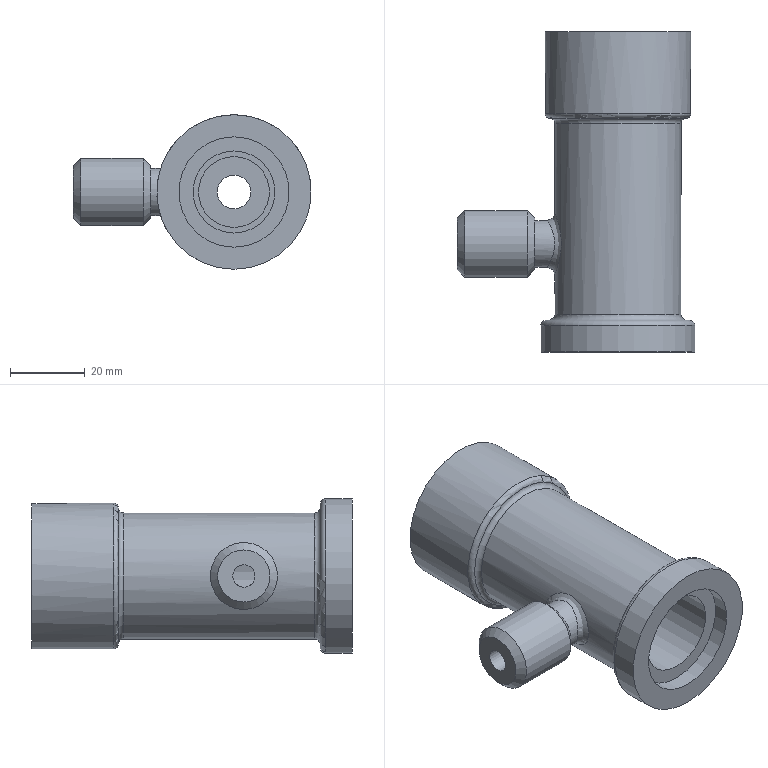Component | NX | VALVE_BODY | 1 solid | 31 faces | volume 56139 mm3 | cylinder 13 | plane 11 | torus 4 | cone 2 | spline 1 | commonest cylinder face diameters 29.6 x2 33.8 x1 39 x1 41.4 x1 22 x1 19 x1 9 x1 23 x1